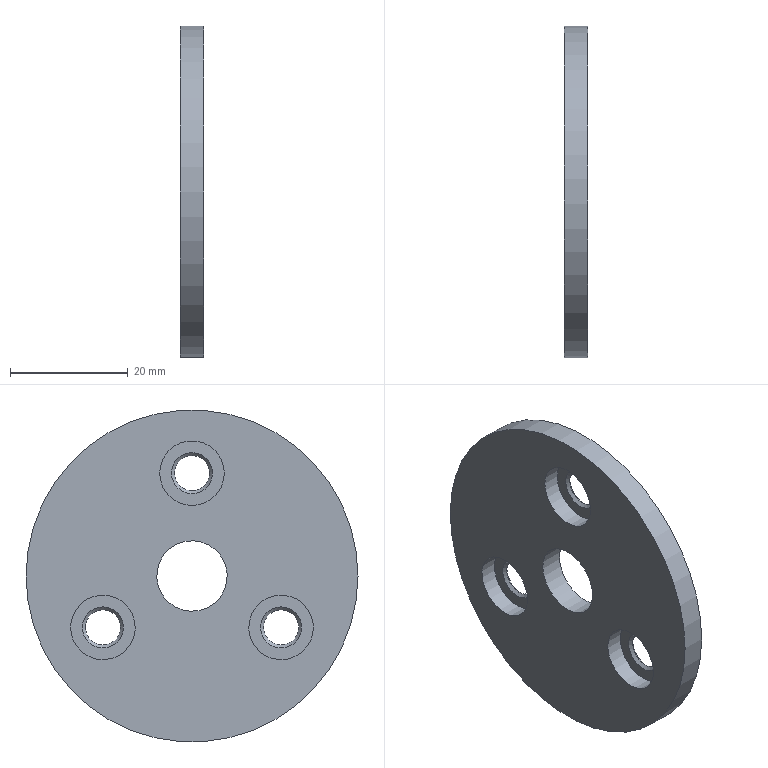Component | NX | FRONT_END_COVER_2 | 1 solid | 16 faces | box 4 x 56.5 x 56.5 mm | volume 8621 mm3 | cone 6 | plane 5 | cylinder 5 | commonest cylinder face diameters 11 x3 56.5 x1 12 x1
STEP:
#1=CARTESIAN_POINT('',(0.,0.,0.));
#2=DIRECTION('',(0.,0.,1.));
#3=DIRECTION('',(1.,0.,0.));
#4=AXIS2_PLACEMENT_3D('',#1,#2,#3);
#5=CARTESIAN_POINT('',(4.,-66.905,79.013));
#6=VERTEX_POINT('',#5);
#7=CARTESIAN_POINT('',(4.,-64.155,74.25));
#8=DIRECTION('',(1.,0.,0.));
#9=DIRECTION('',(0.,-0.5,0.866));
#10=AXIS2_PLACEMENT_3D('',#7,#8,#9);
#11=CIRCLE('',#10,5.5);
#12=CARTESIAN_POINT('',(4.,-49.,83.));
#13=DIRECTION('',(-1.,0.,0.));
#14=DIRECTION('',(0.,-0.5,0.866));
#15=AXIS2_PLACEMENT_3D('',#12,#13,#14);
#16=PLANE('',#15);
#17=CARTESIAN_POINT('',(5.5,-17.5));
#18=CARTESIAN_POINT('',(5.5,-27.026));
#19=CARTESIAN_POINT('',(-2.75,-22.263));
#20=CARTESIAN_POINT('',(-11.,-17.5));
#21=CARTESIAN_POINT('',(-2.75,-12.737));
#22=CARTESIAN_POINT('',(5.5,-7.974));
#23=CARTESIAN_POINT('',(5.5,-17.5));
#24=(BOUNDED_CURVE()B_SPLINE_CURVE(2,(#17,#18,#19,#20,#21,#22,#23),.UNSPECIFIED.,.T.,.F.)B_SPLINE_CURVE_WITH_KNOTS((1,2,2,2,2,1),(-2.094,0.,2.094,4.189,6.283,8.378),.UNSPECIFIED.)CURVE()GEOMETRIC_REPRESENTATION_ITEM()RATIONAL_B_SPLINE_CURVE((1.,0.5,1.,0.5,1.,0.5,1.))REPRESENTATION_ITEM(''));
#25=(GEOMETRIC_REPRESENTATION_CONTEXT(2)PARAMETRIC_REPRESENTATION_CONTEXT()REPRESENTATION_CONTEXT('',''));
#26=DEFINITIONAL_REPRESENTATION('',(#24),#25);
#27=PCURVE('',#16,#26);
#28=CARTESIAN_POINT('',(7.,-64.155,74.25));
#29=DIRECTION('',(-1.,0.,0.));
#30=DIRECTION('',(0.,-0.5,0.866));
#31=AXIS2_PLACEMENT_3D('',#28,#29,#30);
#32=CYLINDRICAL_SURFACE('',#31,5.5);
#33=CARTESIAN_POINT('',(6.283,3.));
#34=DIRECTION('',(-1.,0.));
#35=VECTOR('',#34,1.);
#36=LINE('',#33,#35);
#37=(GEOMETRIC_REPRESENTATION_CONTEXT(2)PARAMETRIC_REPRESENTATION_CONTEXT()REPRESENTATION_CONTEXT('',''));
#38=DEFINITIONAL_REPRESENTATION('',(#36),#37);
#39=PCURVE('',#32,#38);
#40=SURFACE_CURVE('',#11,(#27,#39),.PCURVE_S1.);
#41=EDGE_CURVE('',#6,#6,#40,.T.);
#42=ORIENTED_EDGE('',*,*,#41,.T.);
#43=EDGE_LOOP('',(#42));
#44=FACE_BOUND('',#43,.T.);
#45=CARTESIAN_POINT('',(4.,-36.595,69.487));
#46=VERTEX_POINT('',#45);
#47=CARTESIAN_POINT('',(4.,-33.845,74.25));
#48=DIRECTION('',(1.,0.,0.));
#49=DIRECTION('',(0.,-0.5,-0.866));
#50=AXIS2_PLACEMENT_3D('',#47,#48,#49);
#51=CIRCLE('',#50,5.5);
#52=CARTESIAN_POINT('',(-17.905,3.987));
#53=CARTESIAN_POINT('',(-26.155,8.75));
#54=CARTESIAN_POINT('',(-17.905,13.513));
#55=CARTESIAN_POINT('',(-9.655,18.276));
#56=CARTESIAN_POINT('',(-9.655,8.75));
#57=CARTESIAN_POINT('',(-9.655,-0.7763));
#58=CARTESIAN_POINT('',(-17.905,3.987));
#59=(BOUNDED_CURVE()B_SPLINE_CURVE(2,(#52,#53,#54,#55,#56,#57,#58),.UNSPECIFIED.,.T.,.F.)B_SPLINE_CURVE_WITH_KNOTS((1,2,2,2,2,1),(-2.094,0.,2.094,4.189,6.283,8.378),.UNSPECIFIED.)CURVE()GEOMETRIC_REPRESENTATION_ITEM()RATIONAL_B_SPLINE_CURVE((1.,0.5,1.,0.5,1.,0.5,1.))REPRESENTATION_ITEM(''));
#60=(GEOMETRIC_REPRESENTATION_CONTEXT(2)PARAMETRIC_REPRESENTATION_CONTEXT()REPRESENTATION_CONTEXT('',''));
#61=DEFINITIONAL_REPRESENTATION('',(#59),#60);
#62=PCURVE('',#16,#61);
#63=CARTESIAN_POINT('',(7.,-33.845,74.25));
#64=DIRECTION('',(-1.,0.,0.));
#65=DIRECTION('',(0.,-0.5,0.866));
#66=AXIS2_PLACEMENT_3D('',#63,#64,#65);
#67=CYLINDRICAL_SURFACE('',#66,5.5);
#68=CARTESIAN_POINT('',(10.472,3.));
#69=DIRECTION('',(-1.,0.));
#70=VECTOR('',#69,1.);
#71=LINE('',#68,#70);
#72=(GEOMETRIC_REPRESENTATION_CONTEXT(2)PARAMETRIC_REPRESENTATION_CONTEXT()REPRESENTATION_CONTEXT('',''));
#73=DEFINITIONAL_REPRESENTATION('',(#71),#72);
#74=PCURVE('',#67,#73);
#75=SURFACE_CURVE('',#51,(#62,#74),.PCURVE_S1.);
#76=EDGE_CURVE('',#46,#46,#75,.T.);
#77=ORIENTED_EDGE('',*,*,#76,.T.);
#78=EDGE_LOOP('',(#77));
#79=FACE_BOUND('',#78,.T.);
#80=CARTESIAN_POINT('',(4.,-43.5,100.5));
#81=VERTEX_POINT('',#80);
#82=CARTESIAN_POINT('',(4.,-49.,100.5));
#83=DIRECTION('',(1.,0.,0.));
#84=DIRECTION('',(0.,1.,0.));
#85=AXIS2_PLACEMENT_3D('',#82,#83,#84);
#86=CIRCLE('',#85,5.5);
#87=CARTESIAN_POINT('',(12.405,13.513));
#88=CARTESIAN_POINT('',(20.655,18.276));
#89=CARTESIAN_POINT('',(20.655,8.75));
#90=CARTESIAN_POINT('',(20.655,-0.7763));
#91=CARTESIAN_POINT('',(12.405,3.987));
#92=CARTESIAN_POINT('',(4.155,8.75));
#93=CARTESIAN_POINT('',(12.405,13.513));
#94=(BOUNDED_CURVE()B_SPLINE_CURVE(2,(#87,#88,#89,#90,#91,#92,#93),.UNSPECIFIED.,.T.,.F.)B_SPLINE_CURVE_WITH_KNOTS((1,2,2,2,2,1),(-2.094,0.,2.094,4.189,6.283,8.378),.UNSPECIFIED.)CURVE()GEOMETRIC_REPRESENTATION_ITEM()RATIONAL_B_SPLINE_CURVE((1.,0.5,1.,0.5,1.,0.5,1.))REPRESENTATION_ITEM(''));
#95=(GEOMETRIC_REPRESENTATION_CONTEXT(2)PARAMETRIC_REPRESENTATION_CONTEXT()REPRESENTATION_CONTEXT('',''));
#96=DEFINITIONAL_REPRESENTATION('',(#94),#95);
#97=PCURVE('',#16,#96);
#98=CARTESIAN_POINT('',(7.,-49.,100.5));
#99=DIRECTION('',(-1.,0.,0.));
#100=DIRECTION('',(0.,-0.5,0.866));
#101=AXIS2_PLACEMENT_3D('',#98,#99,#100);
#102=CYLINDRICAL_SURFACE('',#101,5.5);
#103=CARTESIAN_POINT('',(8.378,3.));
#104=DIRECTION('',(-1.,0.));
#105=VECTOR('',#104,1.);
#106=LINE('',#103,#105);
#107=(GEOMETRIC_REPRESENTATION_CONTEXT(2)PARAMETRIC_REPRESENTATION_CONTEXT()REPRESENTATION_CONTEXT('',''));
#108=DEFINITIONAL_REPRESENTATION('',(#106),#107);
#109=PCURVE('',#102,#108);
#110=SURFACE_CURVE('',#86,(#97,#109),.PCURVE_S1.);
#111=EDGE_CURVE('',#81,#81,#110,.T.);
#112=ORIENTED_EDGE('',*,*,#111,.T.);
#113=EDGE_LOOP('',(#112));
#114=FACE_BOUND('',#113,.T.);
#115=CARTESIAN_POINT('',(4.,-52.,88.196));
#116=VERTEX_POINT('',#115);
#117=CARTESIAN_POINT('',(4.,-49.,83.));
#118=DIRECTION('',(-1.,0.,0.));
#119=DIRECTION('',(0.,-0.5,0.866));
#120=AXIS2_PLACEMENT_3D('',#117,#118,#119);
#121=CIRCLE('',#120,6.);
#122=CARTESIAN_POINT('',(0.,0.));
#123=DIRECTION('',(1.,-0.));
#124=AXIS2_PLACEMENT_2D('',#122,#123);
#125=CIRCLE('',#124,6.);
#126=(GEOMETRIC_REPRESENTATION_CONTEXT(2)PARAMETRIC_REPRESENTATION_CONTEXT()REPRESENTATION_CONTEXT('',''));
#127=DEFINITIONAL_REPRESENTATION('',(#125),#126);
#128=PCURVE('',#16,#127);
#129=CARTESIAN_POINT('',(48.,-49.,83.));
#130=DIRECTION('',(-1.,0.,0.));
#131=DIRECTION('',(0.,-0.5,0.866));
#132=AXIS2_PLACEMENT_3D('',#129,#130,#131);
#133=CYLINDRICAL_SURFACE('',#132,6.);
#134=CARTESIAN_POINT('',(0.,44.));
#135=DIRECTION('',(1.,0.));
#136=VECTOR('',#135,1.);
#137=LINE('',#134,#136);
#138=(GEOMETRIC_REPRESENTATION_CONTEXT(2)PARAMETRIC_REPRESENTATION_CONTEXT()REPRESENTATION_CONTEXT('',''));
#139=DEFINITIONAL_REPRESENTATION('',(#137),#138);
#140=PCURVE('',#133,#139);
#141=SURFACE_CURVE('',#121,(#128,#140),.PCURVE_S1.);
#142=EDGE_CURVE('',#116,#116,#141,.T.);
#143=ORIENTED_EDGE('',*,*,#142,.F.);
#144=EDGE_LOOP('',(#143));
#145=FACE_BOUND('',#144,.T.);
#146=CARTESIAN_POINT('',(4.,-63.125,107.465));
#147=VERTEX_POINT('',#146);
#148=CARTESIAN_POINT('',(4.,-49.,83.));
#149=DIRECTION('',(1.,0.,0.));
#150=DIRECTION('',(0.,-0.5,0.866));
#151=AXIS2_PLACEMENT_3D('',#148,#149,#150);
#152=CIRCLE('',#151,28.25);
#153=CARTESIAN_POINT('',(28.25,0.));
#154=CARTESIAN_POINT('',(28.25,-48.93));
#155=CARTESIAN_POINT('',(-14.125,-24.465));
#156=CARTESIAN_POINT('',(-56.5,-0.));
#157=CARTESIAN_POINT('',(-14.125,24.465));
#158=CARTESIAN_POINT('',(28.25,48.93));
#159=CARTESIAN_POINT('',(28.25,0.));
#160=(BOUNDED_CURVE()B_SPLINE_CURVE(2,(#153,#154,#155,#156,#157,#158,#159),.UNSPECIFIED.,.T.,.F.)B_SPLINE_CURVE_WITH_KNOTS((1,2,2,2,2,1),(-2.094,0.,2.094,4.189,6.283,8.378),.UNSPECIFIED.)CURVE()GEOMETRIC_REPRESENTATION_ITEM()RATIONAL_B_SPLINE_CURVE((1.,0.5,1.,0.5,1.,0.5,1.))REPRESENTATION_ITEM(''));
#161=(GEOMETRIC_REPRESENTATION_CONTEXT(2)PARAMETRIC_REPRESENTATION_CONTEXT()REPRESENTATION_CONTEXT('',''));
#162=DEFINITIONAL_REPRESENTATION('',(#160),#161);
#163=PCURVE('',#16,#162);
#164=CARTESIAN_POINT('',(8.,-49.,83.));
#165=DIRECTION('',(-1.,0.,0.));
#166=DIRECTION('',(0.,-0.5,0.866));
#167=AXIS2_PLACEMENT_3D('',#164,#165,#166);
#168=CYLINDRICAL_SURFACE('',#167,28.25);
#169=CARTESIAN_POINT('',(6.283,4.));
#170=DIRECTION('',(-1.,0.));
#171=VECTOR('',#170,1.);
#172=LINE('',#169,#171);
#173=(GEOMETRIC_REPRESENTATION_CONTEXT(2)PARAMETRIC_REPRESENTATION_CONTEXT()REPRESENTATION_CONTEXT('',''));
#174=DEFINITIONAL_REPRESENTATION('',(#172),#173);
#175=PCURVE('',#168,#174);
#176=SURFACE_CURVE('',#152,(#163,#175),.PCURVE_S1.);
#177=EDGE_CURVE('',#147,#147,#176,.T.);
#178=ORIENTED_EDGE('',*,*,#177,.F.);
#179=EDGE_LOOP('',(#178));
#180=FACE_BOUND('',#179,.T.);
#181=ADVANCED_FACE('',(#44,#79,#114,#145,#180),#16,.T.);
#182=CARTESIAN_POINT('',(8.,-47.25,97.469));
#183=VERTEX_POINT('',#182);
#184=CARTESIAN_POINT('',(8.,-49.,100.5));
#185=DIRECTION('',(-1.,0.,0.));
#186=DIRECTION('',(0.,0.5,-0.866));
#187=AXIS2_PLACEMENT_3D('',#184,#185,#186);
#188=CIRCLE('',#187,3.5);
#189=CARTESIAN_POINT('',(8.,-49.,83.));
#190=DIRECTION('',(1.,0.,0.));
#191=DIRECTION('',(0.,0.5,-0.866));
#192=AXIS2_PLACEMENT_3D('',#189,#190,#191);
#193=PLANE('',#192);
#194=CARTESIAN_POINT('',(-11.655,8.75));
#195=CARTESIAN_POINT('',(-11.655,2.688));
#196=CARTESIAN_POINT('',(-16.905,5.719));
#197=CARTESIAN_POINT('',(-22.155,8.75));
#198=CARTESIAN_POINT('',(-16.905,11.781));
#199=CARTESIAN_POINT('',(-11.655,14.812));
#200=CARTESIAN_POINT('',(-11.655,8.75));
#201=(BOUNDED_CURVE()B_SPLINE_CURVE(2,(#194,#195,#196,#197,#198,#199,#200),.UNSPECIFIED.,.T.,.F.)B_SPLINE_CURVE_WITH_KNOTS((1,2,2,2,2,1),(-2.094,0.,2.094,4.189,6.283,8.378),.UNSPECIFIED.)CURVE()GEOMETRIC_REPRESENTATION_ITEM()RATIONAL_B_SPLINE_CURVE((1.,0.5,1.,0.5,1.,0.5,1.))REPRESENTATION_ITEM(''));
#202=(GEOMETRIC_REPRESENTATION_CONTEXT(2)PARAMETRIC_REPRESENTATION_CONTEXT()REPRESENTATION_CONTEXT('',''));
#203=DEFINITIONAL_REPRESENTATION('',(#201),#202);
#204=PCURVE('',#193,#203);
#205=CARTESIAN_POINT('',(7.5,-49.,100.5));
#206=DIRECTION('',(1.,0.,0.));
#207=DIRECTION('',(0.,0.5,-0.866));
#208=AXIS2_PLACEMENT_3D('',#205,#206,#207);
#209=CONICAL_SURFACE('',#208,3.,0.7854);
#210=CARTESIAN_POINT('',(6.283,0.5));
#211=DIRECTION('',(-1.,0.));
#212=VECTOR('',#211,1.);
#213=LINE('',#210,#212);
#214=(GEOMETRIC_REPRESENTATION_CONTEXT(2)PARAMETRIC_REPRESENTATION_CONTEXT()REPRESENTATION_CONTEXT('',''));
#215=DEFINITIONAL_REPRESENTATION('',(#213),#214);
#216=PCURVE('',#209,#215);
#217=SURFACE_CURVE('',#188,(#204,#216),.PCURVE_S1.);
#218=EDGE_CURVE('',#183,#183,#217,.T.);
#219=ORIENTED_EDGE('',*,*,#218,.T.);
#220=EDGE_LOOP('',(#219));
#221=FACE_BOUND('',#220,.T.);
#222=CARTESIAN_POINT('',(8.,-62.405,71.219));
#223=VERTEX_POINT('',#222);
#224=CARTESIAN_POINT('',(8.,-64.155,74.25));
#225=DIRECTION('',(-1.,0.,0.));
#226=DIRECTION('',(0.,0.5,-0.866));
#227=AXIS2_PLACEMENT_3D('',#224,#225,#226);
#228=CIRCLE('',#227,3.5);
#229=CARTESIAN_POINT('',(3.5,-17.5));
#230=CARTESIAN_POINT('',(3.5,-23.562));
#231=CARTESIAN_POINT('',(-1.75,-20.531));
#232=CARTESIAN_POINT('',(-7.,-17.5));
#233=CARTESIAN_POINT('',(-1.75,-14.469));
#234=CARTESIAN_POINT('',(3.5,-11.438));
#235=CARTESIAN_POINT('',(3.5,-17.5));
#236=(BOUNDED_CURVE()B_SPLINE_CURVE(2,(#229,#230,#231,#232,#233,#234,#235),.UNSPECIFIED.,.T.,.F.)B_SPLINE_CURVE_WITH_KNOTS((1,2,2,2,2,1),(-2.094,0.,2.094,4.189,6.283,8.378),.UNSPECIFIED.)CURVE()GEOMETRIC_REPRESENTATION_ITEM()RATIONAL_B_SPLINE_CURVE((1.,0.5,1.,0.5,1.,0.5,1.))REPRESENTATION_ITEM(''));
#237=(GEOMETRIC_REPRESENTATION_CONTEXT(2)PARAMETRIC_REPRESENTATION_CONTEXT()REPRESENTATION_CONTEXT('',''));
#238=DEFINITIONAL_REPRESENTATION('',(#236),#237);
#239=PCURVE('',#193,#238);
#240=CARTESIAN_POINT('',(7.5,-64.155,74.25));
#241=DIRECTION('',(1.,0.,0.));
#242=DIRECTION('',(0.,0.5,-0.866));
#243=AXIS2_PLACEMENT_3D('',#240,#241,#242);
#244=CONICAL_SURFACE('',#243,3.,0.7854);
#245=CARTESIAN_POINT('',(6.283,0.5));
#246=DIRECTION('',(-1.,0.));
#247=VECTOR('',#246,1.);
#248=LINE('',#245,#247);
#249=(GEOMETRIC_REPRESENTATION_CONTEXT(2)PARAMETRIC_REPRESENTATION_CONTEXT()REPRESENTATION_CONTEXT('',''));
#250=DEFINITIONAL_REPRESENTATION('',(#248),#249);
#251=PCURVE('',#244,#250);
#252=SURFACE_CURVE('',#228,(#239,#251),.PCURVE_S1.);
#253=EDGE_CURVE('',#223,#223,#252,.T.);
#254=ORIENTED_EDGE('',*,*,#253,.T.);
#255=EDGE_LOOP('',(#254));
#256=FACE_BOUND('',#255,.T.);
#257=CARTESIAN_POINT('',(8.,-32.095,71.219));
#258=VERTEX_POINT('',#257);
#259=CARTESIAN_POINT('',(8.,-33.845,74.25));
#260=DIRECTION('',(-1.,0.,0.));
#261=DIRECTION('',(0.,0.5,-0.866));
#262=AXIS2_PLACEMENT_3D('',#259,#260,#261);
#263=CIRCLE('',#262,3.5);
#264=CARTESIAN_POINT('',(18.655,8.75));
#265=CARTESIAN_POINT('',(18.655,2.688));
#266=CARTESIAN_POINT('',(13.405,5.719));
#267=CARTESIAN_POINT('',(8.155,8.75));
#268=CARTESIAN_POINT('',(13.405,11.781));
#269=CARTESIAN_POINT('',(18.655,14.812));
#270=CARTESIAN_POINT('',(18.655,8.75));
#271=(BOUNDED_CURVE()B_SPLINE_CURVE(2,(#264,#265,#266,#267,#268,#269,#270),.UNSPECIFIED.,.T.,.F.)B_SPLINE_CURVE_WITH_KNOTS((1,2,2,2,2,1),(-2.094,0.,2.094,4.189,6.283,8.378),.UNSPECIFIED.)CURVE()GEOMETRIC_REPRESENTATION_ITEM()RATIONAL_B_SPLINE_CURVE((1.,0.5,1.,0.5,1.,0.5,1.))REPRESENTATION_ITEM(''));
#272=(GEOMETRIC_REPRESENTATION_CONTEXT(2)PARAMETRIC_REPRESENTATION_CONTEXT()REPRESENTATION_CONTEXT('',''));
#273=DEFINITIONAL_REPRESENTATION('',(#271),#272);
#274=PCURVE('',#193,#273);
#275=CARTESIAN_POINT('',(7.5,-33.845,74.25));
#276=DIRECTION('',(1.,0.,0.));
#277=DIRECTION('',(0.,0.5,-0.866));
#278=AXIS2_PLACEMENT_3D('',#275,#276,#277);
#279=CONICAL_SURFACE('',#278,3.,0.7854);
#280=CARTESIAN_POINT('',(6.283,0.5));
#281=DIRECTION('',(-1.,-0.));
#282=VECTOR('',#281,1.);
#283=LINE('',#280,#282);
#284=(GEOMETRIC_REPRESENTATION_CONTEXT(2)PARAMETRIC_REPRESENTATION_CONTEXT()REPRESENTATION_CONTEXT('',''));
#285=DEFINITIONAL_REPRESENTATION('',(#283),#284);
#286=PCURVE('',#279,#285);
#287=SURFACE_CURVE('',#263,(#274,#286),.PCURVE_S1.);
#288=EDGE_CURVE('',#258,#258,#287,.T.);
#289=ORIENTED_EDGE('',*,*,#288,.T.);
#290=EDGE_LOOP('',(#289));
#291=FACE_BOUND('',#290,.T.);
#292=CARTESIAN_POINT('',(8.,-46.,77.804));
#293=VERTEX_POINT('',#292);
#294=CARTESIAN_POINT('',(8.,-52.,88.196));
#295=VERTEX_POINT('',#294);
#296=CARTESIAN_POINT('',(8.,-49.,83.));
#297=DIRECTION('',(1.,0.,0.));
#298=DIRECTION('',(0.,0.5,-0.866));
#299=AXIS2_PLACEMENT_3D('',#296,#297,#298);
#300=CIRCLE('',#299,6.);
#301=CARTESIAN_POINT('',(0.,0.));
#302=DIRECTION('',(1.,0.));
#303=AXIS2_PLACEMENT_2D('',#301,#302);
#304=CIRCLE('',#303,6.);
#305=(GEOMETRIC_REPRESENTATION_CONTEXT(2)PARAMETRIC_REPRESENTATION_CONTEXT()REPRESENTATION_CONTEXT('',''));
#306=DEFINITIONAL_REPRESENTATION('',(#304),#305);
#307=PCURVE('',#193,#306);
#308=CARTESIAN_POINT('',(3.142,40.));
#309=DIRECTION('',(-1.,0.));
#310=VECTOR('',#309,1.);
#311=LINE('',#308,#310);
#312=(GEOMETRIC_REPRESENTATION_CONTEXT(2)PARAMETRIC_REPRESENTATION_CONTEXT()REPRESENTATION_CONTEXT('',''));
#313=DEFINITIONAL_REPRESENTATION('',(#311),#312);
#314=PCURVE('',#133,#313);
#315=SURFACE_CURVE('',#300,(#307,#314),.PCURVE_S1.);
#316=EDGE_CURVE('',#293,#295,#315,.T.);
#317=ORIENTED_EDGE('',*,*,#316,.F.);
#318=CARTESIAN_POINT('',(8.,-49.,83.));
#319=DIRECTION('',(1.,0.,0.));
#320=DIRECTION('',(0.,0.5,-0.866));
#321=AXIS2_PLACEMENT_3D('',#318,#319,#320);
#322=CIRCLE('',#321,6.);
#323=CARTESIAN_POINT('',(0.,0.));
#324=DIRECTION('',(1.,0.));
#325=AXIS2_PLACEMENT_2D('',#323,#324);
#326=CIRCLE('',#325,6.);
#327=(GEOMETRIC_REPRESENTATION_CONTEXT(2)PARAMETRIC_REPRESENTATION_CONTEXT()REPRESENTATION_CONTEXT('',''));
#328=DEFINITIONAL_REPRESENTATION('',(#326),#327);
#329=PCURVE('',#193,#328);
#330=CARTESIAN_POINT('',(9.425,40.));
#331=DIRECTION('',(-1.,0.));
#332=VECTOR('',#331,1.);
#333=LINE('',#330,#332);
#334=(GEOMETRIC_REPRESENTATION_CONTEXT(2)PARAMETRIC_REPRESENTATION_CONTEXT()REPRESENTATION_CONTEXT('',''));
#335=DEFINITIONAL_REPRESENTATION('',(#333),#334);
#336=PCURVE('',#133,#335);
#337=SURFACE_CURVE('',#322,(#329,#336),.PCURVE_S1.);
#338=EDGE_CURVE('',#295,#293,#337,.T.);
#339=ORIENTED_EDGE('',*,*,#338,.F.);
#340=EDGE_LOOP('',(#317,#339));
#341=FACE_BOUND('',#340,.T.);
#342=CARTESIAN_POINT('',(8.,-63.125,107.465));
#343=VERTEX_POINT('',#342);
#344=CARTESIAN_POINT('',(8.,-49.,83.));
#345=DIRECTION('',(-1.,0.,0.));
#346=DIRECTION('',(0.,-0.5,0.866));
#347=AXIS2_PLACEMENT_3D('',#344,#345,#346);
#348=CIRCLE('',#347,28.25);
#349=CARTESIAN_POINT('',(-28.25,0.));
#350=CARTESIAN_POINT('',(-28.25,48.93));
#351=CARTESIAN_POINT('',(14.125,24.465));
#352=CARTESIAN_POINT('',(56.5,0.));
#353=CARTESIAN_POINT('',(14.125,-24.465));
#354=CARTESIAN_POINT('',(-28.25,-48.93));
#355=CARTESIAN_POINT('',(-28.25,0.));
#356=(BOUNDED_CURVE()B_SPLINE_CURVE(2,(#349,#350,#351,#352,#353,#354,#355),.UNSPECIFIED.,.T.,.F.)B_SPLINE_CURVE_WITH_KNOTS((1,2,2,2,2,1),(-2.094,0.,2.094,4.189,6.283,8.378),.UNSPECIFIED.)CURVE()GEOMETRIC_REPRESENTATION_ITEM()RATIONAL_B_SPLINE_CURVE((1.,0.5,1.,0.5,1.,0.5,1.))REPRESENTATION_ITEM(''));
#357=(GEOMETRIC_REPRESENTATION_CONTEXT(2)PARAMETRIC_REPRESENTATION_CONTEXT()REPRESENTATION_CONTEXT('',''));
#358=DEFINITIONAL_REPRESENTATION('',(#356),#357);
#359=PCURVE('',#193,#358);
#360=CARTESIAN_POINT('',(0.,0.));
#361=DIRECTION('',(1.,0.));
#362=VECTOR('',#361,1.);
#363=LINE('',#360,#362);
#364=(GEOMETRIC_REPRESENTATION_CONTEXT(2)PARAMETRIC_REPRESENTATION_CONTEXT()REPRESENTATION_CONTEXT('',''));
#365=DEFINITIONAL_REPRESENTATION('',(#363),#364);
#366=PCURVE('',#168,#365);
#367=SURFACE_CURVE('',#348,(#359,#366),.PCURVE_S1.);
#368=EDGE_CURVE('',#343,#343,#367,.T.);
#369=ORIENTED_EDGE('',*,*,#368,.F.);
#370=EDGE_LOOP('',(#369));
#371=FACE_BOUND('',#370,.T.);
#372=ADVANCED_FACE('',(#221,#256,#291,#341,#371),#193,.T.);
#373=ORIENTED_EDGE('',*,*,#177,.T.);
#374=CARTESIAN_POINT('',(8.,-63.125,107.465));
#375=CARTESIAN_POINT('',(4.,-63.125,107.465));
#376=B_SPLINE_CURVE_WITH_KNOTS('',1,(#374,#375),.UNSPECIFIED.,.F.,.F.,(2,2),(0.,4.),.PIECEWISE_BEZIER_KNOTS.);
#377=CARTESIAN_POINT('',(0.,0.));
#378=DIRECTION('',(0.,1.));
#379=VECTOR('',#378,1.);
#380=LINE('',#377,#379);
#381=(GEOMETRIC_REPRESENTATION_CONTEXT(2)PARAMETRIC_REPRESENTATION_CONTEXT()REPRESENTATION_CONTEXT('',''));
#382=DEFINITIONAL_REPRESENTATION('',(#380),#381);
#383=PCURVE('',#168,#382);
#384=CARTESIAN_POINT('',(6.283,0.));
#385=DIRECTION('',(0.,1.));
#386=VECTOR('',#385,1.);
#387=LINE('',#384,#386);
#388=(GEOMETRIC_REPRESENTATION_CONTEXT(2)PARAMETRIC_REPRESENTATION_CONTEXT()REPRESENTATION_CONTEXT('',''));
#389=DEFINITIONAL_REPRESENTATION('',(#387),#388);
#390=PCURVE('',#168,#389);
#391=SEAM_CURVE('',#376,(#383,#390),.PCURVE_S1.);
#392=EDGE_CURVE('',#343,#147,#391,.T.);
#393=ORIENTED_EDGE('',*,*,#392,.F.);
#394=ORIENTED_EDGE('',*,*,#368,.T.);
#395=ORIENTED_EDGE('',*,*,#392,.T.);
#396=EDGE_LOOP('',(#373,#393,#394,#395));
#397=FACE_BOUND('',#396,.T.);
#398=ADVANCED_FACE('',(#397),#168,.T.);
#399=ORIENTED_EDGE('',*,*,#338,.F.);
#400=CARTESIAN_POINT('',(8.,-52.,88.196));
#401=CARTESIAN_POINT('',(4.,-52.,88.196));
#402=B_SPLINE_CURVE_WITH_KNOTS('',1,(#400,#401),.UNSPECIFIED.,.F.,.F.,(2,2),(40.,44.),.PIECEWISE_BEZIER_KNOTS.);
#403=CARTESIAN_POINT('',(6.283,0.));
#404=DIRECTION('',(0.,1.));
#405=VECTOR('',#404,1.);
#406=LINE('',#403,#405);
#407=(GEOMETRIC_REPRESENTATION_CONTEXT(2)PARAMETRIC_REPRESENTATION_CONTEXT()REPRESENTATION_CONTEXT('',''));
#408=DEFINITIONAL_REPRESENTATION('',(#406),#407);
#409=PCURVE('',#133,#408);
#410=CARTESIAN_POINT('',(0.,0.));
#411=DIRECTION('',(0.,1.));
#412=VECTOR('',#411,1.);
#413=LINE('',#410,#412);
#414=(GEOMETRIC_REPRESENTATION_CONTEXT(2)PARAMETRIC_REPRESENTATION_CONTEXT()REPRESENTATION_CONTEXT('',''));
#415=DEFINITIONAL_REPRESENTATION('',(#413),#414);
#416=PCURVE('',#133,#415);
#417=SEAM_CURVE('',#402,(#409,#416),.PCURVE_S1.);
#418=EDGE_CURVE('',#295,#116,#417,.T.);
#419=ORIENTED_EDGE('',*,*,#418,.T.);
#420=ORIENTED_EDGE('',*,*,#142,.F.);
#421=ORIENTED_EDGE('',*,*,#418,.F.);
#422=ORIENTED_EDGE('',*,*,#316,.F.);
#423=EDGE_LOOP('',(#399,#419,#420,#421,#422));
#424=FACE_BOUND('',#423,.F.);
#425=ADVANCED_FACE('',(#424),#133,.F.);
#426=CARTESIAN_POINT('',(7.,-43.5,100.5));
#427=VERTEX_POINT('',#426);
#428=CARTESIAN_POINT('',(7.,-49.,100.5));
#429=DIRECTION('',(-1.,0.,0.));
#430=DIRECTION('',(0.,1.,0.));
#431=AXIS2_PLACEMENT_3D('',#428,#429,#430);
#432=CIRCLE('',#431,5.5);
#433=CARTESIAN_POINT('',(2.094,0.));
#434=DIRECTION('',(1.,0.));
#435=VECTOR('',#434,1.);
#436=LINE('',#433,#435);
#437=(GEOMETRIC_REPRESENTATION_CONTEXT(2)PARAMETRIC_REPRESENTATION_CONTEXT()REPRESENTATION_CONTEXT('',''));
#438=DEFINITIONAL_REPRESENTATION('',(#436),#437);
#439=PCURVE('',#102,#438);
#440=CARTESIAN_POINT('',(7.,-49.,100.5));
#441=DIRECTION('',(1.,0.,0.));
#442=DIRECTION('',(0.,0.5,-0.866));
#443=AXIS2_PLACEMENT_3D('',#440,#441,#442);
#444=PLANE('',#443);
#445=CARTESIAN_POINT('',(2.75,4.763));
#446=CARTESIAN_POINT('',(11.,0.));
#447=CARTESIAN_POINT('',(2.75,-4.763));
#448=CARTESIAN_POINT('',(-5.5,-9.526));
#449=CARTESIAN_POINT('',(-5.5,-0.));
#450=CARTESIAN_POINT('',(-5.5,9.526));
#451=CARTESIAN_POINT('',(2.75,4.763));
#452=(BOUNDED_CURVE()B_SPLINE_CURVE(2,(#445,#446,#447,#448,#449,#450,#451),.UNSPECIFIED.,.T.,.F.)B_SPLINE_CURVE_WITH_KNOTS((1,2,2,2,2,1),(-2.094,0.,2.094,4.189,6.283,8.378),.UNSPECIFIED.)CURVE()GEOMETRIC_REPRESENTATION_ITEM()RATIONAL_B_SPLINE_CURVE((1.,0.5,1.,0.5,1.,0.5,1.))REPRESENTATION_ITEM(''));
#453=(GEOMETRIC_REPRESENTATION_CONTEXT(2)PARAMETRIC_REPRESENTATION_CONTEXT()REPRESENTATION_CONTEXT('',''));
#454=DEFINITIONAL_REPRESENTATION('',(#452),#453);
#455=PCURVE('',#444,#454);
#456=SURFACE_CURVE('',#432,(#439,#455),.PCURVE_S1.);
#457=EDGE_CURVE('',#427,#427,#456,.T.);
#458=ORIENTED_EDGE('',*,*,#457,.T.);
#459=CARTESIAN_POINT('',(7.,-43.5,100.5));
#460=CARTESIAN_POINT('',(4.,-43.5,100.5));
#461=B_SPLINE_CURVE_WITH_KNOTS('',1,(#459,#460),.UNSPECIFIED.,.F.,.F.,(2,2),(0.,3.),.PIECEWISE_BEZIER_KNOTS.);
#462=CARTESIAN_POINT('',(8.378,0.));
#463=DIRECTION('',(0.,1.));
#464=VECTOR('',#463,1.);
#465=LINE('',#462,#464);
#466=(GEOMETRIC_REPRESENTATION_CONTEXT(2)PARAMETRIC_REPRESENTATION_CONTEXT()REPRESENTATION_CONTEXT('',''));
#467=DEFINITIONAL_REPRESENTATION('',(#465),#466);
#468=PCURVE('',#102,#467);
#469=CARTESIAN_POINT('',(2.094,0.));
#470=DIRECTION('',(0.,1.));
#471=VECTOR('',#470,1.);
#472=LINE('',#469,#471);
#473=(GEOMETRIC_REPRESENTATION_CONTEXT(2)PARAMETRIC_REPRESENTATION_CONTEXT()REPRESENTATION_CONTEXT('',''));
#474=DEFINITIONAL_REPRESENTATION('',(#472),#473);
#475=PCURVE('',#102,#474);
#476=SEAM_CURVE('',#461,(#468,#475),.PCURVE_S1.);
#477=EDGE_CURVE('',#427,#81,#476,.T.);
#478=ORIENTED_EDGE('',*,*,#477,.T.);
#479=ORIENTED_EDGE('',*,*,#111,.T.);
#480=ORIENTED_EDGE('',*,*,#477,.F.);
#481=EDGE_LOOP('',(#458,#478,#479,#480));
#482=FACE_BOUND('',#481,.F.);
#483=ADVANCED_FACE('',(#482),#102,.F.);
#484=CARTESIAN_POINT('',(7.,-47.25,97.469));
#485=VERTEX_POINT('',#484);
#486=CARTESIAN_POINT('',(7.,-49.,100.5));
#487=DIRECTION('',(1.,0.,0.));
#488=DIRECTION('',(0.,0.5,-0.866));
#489=AXIS2_PLACEMENT_3D('',#486,#487,#488);
#490=CIRCLE('',#489,3.5);
#491=CARTESIAN_POINT('',(0.,0.));
#492=DIRECTION('',(1.,-0.));
#493=AXIS2_PLACEMENT_2D('',#491,#492);
#494=CIRCLE('',#493,3.5);
#495=(GEOMETRIC_REPRESENTATION_CONTEXT(2)PARAMETRIC_REPRESENTATION_CONTEXT()REPRESENTATION_CONTEXT('',''));
#496=DEFINITIONAL_REPRESENTATION('',(#494),#495);
#497=PCURVE('',#444,#496);
#498=CARTESIAN_POINT('',(7.,-49.,100.5));
#499=DIRECTION('',(-1.,0.,0.));
#500=DIRECTION('',(0.,-0.5,0.866));
#501=AXIS2_PLACEMENT_3D('',#498,#499,#500);
#502=CONICAL_SURFACE('',#501,3.5,0.7854);
#503=CARTESIAN_POINT('',(9.425,0.));
#504=DIRECTION('',(-1.,0.));
#505=VECTOR('',#504,1.);
#506=LINE('',#503,#505);
#507=(GEOMETRIC_REPRESENTATION_CONTEXT(2)PARAMETRIC_REPRESENTATION_CONTEXT()REPRESENTATION_CONTEXT('',''));
#508=DEFINITIONAL_REPRESENTATION('',(#506),#507);
#509=PCURVE('',#502,#508);
#510=SURFACE_CURVE('',#490,(#497,#509),.PCURVE_S1.);
#511=EDGE_CURVE('',#485,#485,#510,.T.);
#512=ORIENTED_EDGE('',*,*,#511,.T.);
#513=EDGE_LOOP('',(#512));
#514=FACE_BOUND('',#513,.T.);
#515=ORIENTED_EDGE('',*,*,#457,.T.);
#516=EDGE_LOOP('',(#515));
#517=FACE_BOUND('',#516,.T.);
#518=ADVANCED_FACE('',(#514,#517),#444,.F.);
#519=CARTESIAN_POINT('',(7.,-36.595,69.487));
#520=VERTEX_POINT('',#519);
#521=CARTESIAN_POINT('',(7.,-33.845,74.25));
#522=DIRECTION('',(-1.,0.,0.));
#523=DIRECTION('',(0.,-0.5,-0.866));
#524=AXIS2_PLACEMENT_3D('',#521,#522,#523);
#525=CIRCLE('',#524,5.5);
#526=CARTESIAN_POINT('',(4.189,0.));
#527=DIRECTION('',(1.,0.));
#528=VECTOR('',#527,1.);
#529=LINE('',#526,#528);
#530=(GEOMETRIC_REPRESENTATION_CONTEXT(2)PARAMETRIC_REPRESENTATION_CONTEXT()REPRESENTATION_CONTEXT('',''));
#531=DEFINITIONAL_REPRESENTATION('',(#529),#530);
#532=PCURVE('',#67,#531);
#533=CARTESIAN_POINT('',(7.,-33.845,74.25));
#534=DIRECTION('',(1.,0.,0.));
#535=DIRECTION('',(0.,0.5,-0.866));
#536=AXIS2_PLACEMENT_3D('',#533,#534,#535);
#537=PLANE('',#536);
#538=CARTESIAN_POINT('',(2.75,-4.763));
#539=CARTESIAN_POINT('',(-5.5,-9.526));
#540=CARTESIAN_POINT('',(-5.5,-0.));
#541=CARTESIAN_POINT('',(-5.5,9.526));
#542=CARTESIAN_POINT('',(2.75,4.763));
#543=CARTESIAN_POINT('',(11.,0.));
#544=CARTESIAN_POINT('',(2.75,-4.763));
#545=(BOUNDED_CURVE()B_SPLINE_CURVE(2,(#538,#539,#540,#541,#542,#543,#544),.UNSPECIFIED.,.T.,.F.)B_SPLINE_CURVE_WITH_KNOTS((1,2,2,2,2,1),(-2.094,0.,2.094,4.189,6.283,8.378),.UNSPECIFIED.)CURVE()GEOMETRIC_REPRESENTATION_ITEM()RATIONAL_B_SPLINE_CURVE((1.,0.5,1.,0.5,1.,0.5,1.))REPRESENTATION_ITEM(''));
#546=(GEOMETRIC_REPRESENTATION_CONTEXT(2)PARAMETRIC_REPRESENTATION_CONTEXT()REPRESENTATION_CONTEXT('',''));
#547=DEFINITIONAL_REPRESENTATION('',(#545),#546);
#548=PCURVE('',#537,#547);
#549=SURFACE_CURVE('',#525,(#532,#548),.PCURVE_S1.);
#550=EDGE_CURVE('',#520,#520,#549,.T.);
#551=ORIENTED_EDGE('',*,*,#550,.T.);
#552=CARTESIAN_POINT('',(7.,-36.595,69.487));
#553=CARTESIAN_POINT('',(4.,-36.595,69.487));
#554=B_SPLINE_CURVE_WITH_KNOTS('',1,(#552,#553),.UNSPECIFIED.,.F.,.F.,(2,2),(0.,3.),.PIECEWISE_BEZIER_KNOTS.);
#555=CARTESIAN_POINT('',(10.472,0.));
#556=DIRECTION('',(0.,1.));
#557=VECTOR('',#556,1.);
#558=LINE('',#555,#557);
#559=(GEOMETRIC_REPRESENTATION_CONTEXT(2)PARAMETRIC_REPRESENTATION_CONTEXT()REPRESENTATION_CONTEXT('',''));
#560=DEFINITIONAL_REPRESENTATION('',(#558),#559);
#561=PCURVE('',#67,#560);
#562=CARTESIAN_POINT('',(4.189,0.));
#563=DIRECTION('',(0.,1.));
#564=VECTOR('',#563,1.);
#565=LINE('',#562,#564);
#566=(GEOMETRIC_REPRESENTATION_CONTEXT(2)PARAMETRIC_REPRESENTATION_CONTEXT()REPRESENTATION_CONTEXT('',''));
#567=DEFINITIONAL_REPRESENTATION('',(#565),#566);
#568=PCURVE('',#67,#567);
#569=SEAM_CURVE('',#554,(#561,#568),.PCURVE_S1.);
#570=EDGE_CURVE('',#520,#46,#569,.T.);
#571=ORIENTED_EDGE('',*,*,#570,.T.);
#572=ORIENTED_EDGE('',*,*,#76,.T.);
#573=ORIENTED_EDGE('',*,*,#570,.F.);
#574=EDGE_LOOP('',(#551,#571,#572,#573));
#575=FACE_BOUND('',#574,.F.);
#576=ADVANCED_FACE('',(#575),#67,.F.);
#577=CARTESIAN_POINT('',(7.,-32.095,71.219));
#578=VERTEX_POINT('',#577);
#579=CARTESIAN_POINT('',(7.,-33.845,74.25));
#580=DIRECTION('',(1.,0.,0.));
#581=DIRECTION('',(0.,0.5,-0.866));
#582=AXIS2_PLACEMENT_3D('',#579,#580,#581);
#583=CIRCLE('',#582,3.5);
#584=CARTESIAN_POINT('',(0.,0.));
#585=DIRECTION('',(1.,-0.));
#586=AXIS2_PLACEMENT_2D('',#584,#585);
#587=CIRCLE('',#586,3.5);
#588=(GEOMETRIC_REPRESENTATION_CONTEXT(2)PARAMETRIC_REPRESENTATION_CONTEXT()REPRESENTATION_CONTEXT('',''));
#589=DEFINITIONAL_REPRESENTATION('',(#587),#588);
#590=PCURVE('',#537,#589);
#591=CARTESIAN_POINT('',(7.,-33.845,74.25));
#592=DIRECTION('',(-1.,0.,0.));
#593=DIRECTION('',(0.,-0.5,0.866));
#594=AXIS2_PLACEMENT_3D('',#591,#592,#593);
#595=CONICAL_SURFACE('',#594,3.5,0.7854);
#596=CARTESIAN_POINT('',(9.425,0.));
#597=DIRECTION('',(-1.,0.));
#598=VECTOR('',#597,1.);
#599=LINE('',#596,#598);
#600=(GEOMETRIC_REPRESENTATION_CONTEXT(2)PARAMETRIC_REPRESENTATION_CONTEXT()REPRESENTATION_CONTEXT('',''));
#601=DEFINITIONAL_REPRESENTATION('',(#599),#600);
#602=PCURVE('',#595,#601);
#603=SURFACE_CURVE('',#583,(#590,#602),.PCURVE_S1.);
#604=EDGE_CURVE('',#578,#578,#603,.T.);
#605=ORIENTED_EDGE('',*,*,#604,.T.);
#606=EDGE_LOOP('',(#605));
#607=FACE_BOUND('',#606,.T.);
#608=ORIENTED_EDGE('',*,*,#550,.T.);
#609=EDGE_LOOP('',(#608));
#610=FACE_BOUND('',#609,.T.);
#611=ADVANCED_FACE('',(#607,#610),#537,.F.);
#612=CARTESIAN_POINT('',(7.,-66.905,79.013));
#613=VERTEX_POINT('',#612);
#614=CARTESIAN_POINT('',(7.,-64.155,74.25));
#615=DIRECTION('',(-1.,0.,0.));
#616=DIRECTION('',(0.,-0.5,0.866));
#617=AXIS2_PLACEMENT_3D('',#614,#615,#616);
#618=CIRCLE('',#617,5.5);
#619=CARTESIAN_POINT('',(0.,0.));
#620=DIRECTION('',(1.,0.));
#621=VECTOR('',#620,1.);
#622=LINE('',#619,#621);
#623=(GEOMETRIC_REPRESENTATION_CONTEXT(2)PARAMETRIC_REPRESENTATION_CONTEXT()REPRESENTATION_CONTEXT('',''));
#624=DEFINITIONAL_REPRESENTATION('',(#622),#623);
#625=PCURVE('',#32,#624);
#626=CARTESIAN_POINT('',(7.,-64.155,74.25));
#627=DIRECTION('',(1.,0.,0.));
#628=DIRECTION('',(0.,0.5,-0.866));
#629=AXIS2_PLACEMENT_3D('',#626,#627,#628);
#630=PLANE('',#629);
#631=CARTESIAN_POINT('',(-5.5,0.));
#632=CARTESIAN_POINT('',(-5.5,9.526));
#633=CARTESIAN_POINT('',(2.75,4.763));
#634=CARTESIAN_POINT('',(11.,-0.));
#635=CARTESIAN_POINT('',(2.75,-4.763));
#636=CARTESIAN_POINT('',(-5.5,-9.526));
#637=CARTESIAN_POINT('',(-5.5,0.));
#638=(BOUNDED_CURVE()B_SPLINE_CURVE(2,(#631,#632,#633,#634,#635,#636,#637),.UNSPECIFIED.,.T.,.F.)B_SPLINE_CURVE_WITH_KNOTS((1,2,2,2,2,1),(-2.094,0.,2.094,4.189,6.283,8.378),.UNSPECIFIED.)CURVE()GEOMETRIC_REPRESENTATION_ITEM()RATIONAL_B_SPLINE_CURVE((1.,0.5,1.,0.5,1.,0.5,1.))REPRESENTATION_ITEM(''));
#639=(GEOMETRIC_REPRESENTATION_CONTEXT(2)PARAMETRIC_REPRESENTATION_CONTEXT()REPRESENTATION_CONTEXT('',''));
#640=DEFINITIONAL_REPRESENTATION('',(#638),#639);
#641=PCURVE('',#630,#640);
#642=SURFACE_CURVE('',#618,(#625,#641),.PCURVE_S1.);
#643=EDGE_CURVE('',#613,#613,#642,.T.);
#644=ORIENTED_EDGE('',*,*,#643,.T.);
#645=CARTESIAN_POINT('',(7.,-66.905,79.013));
#646=CARTESIAN_POINT('',(4.,-66.905,79.013));
#647=B_SPLINE_CURVE_WITH_KNOTS('',1,(#645,#646),.UNSPECIFIED.,.F.,.F.,(2,2),(0.,3.),.PIECEWISE_BEZIER_KNOTS.);
#648=CARTESIAN_POINT('',(6.283,0.));
#649=DIRECTION('',(0.,1.));
#650=VECTOR('',#649,1.);
#651=LINE('',#648,#650);
#652=(GEOMETRIC_REPRESENTATION_CONTEXT(2)PARAMETRIC_REPRESENTATION_CONTEXT()REPRESENTATION_CONTEXT('',''));
#653=DEFINITIONAL_REPRESENTATION('',(#651),#652);
#654=PCURVE('',#32,#653);
#655=CARTESIAN_POINT('',(0.,0.));
#656=DIRECTION('',(0.,1.));
#657=VECTOR('',#656,1.);
#658=LINE('',#655,#657);
#659=(GEOMETRIC_REPRESENTATION_CONTEXT(2)PARAMETRIC_REPRESENTATION_CONTEXT()REPRESENTATION_CONTEXT('',''));
#660=DEFINITIONAL_REPRESENTATION('',(#658),#659);
#661=PCURVE('',#32,#660);
#662=SEAM_CURVE('',#647,(#654,#661),.PCURVE_S1.);
#663=EDGE_CURVE('',#613,#6,#662,.T.);
#664=ORIENTED_EDGE('',*,*,#663,.T.);
#665=ORIENTED_EDGE('',*,*,#41,.T.);
#666=ORIENTED_EDGE('',*,*,#663,.F.);
#667=EDGE_LOOP('',(#644,#664,#665,#666));
#668=FACE_BOUND('',#667,.F.);
#669=ADVANCED_FACE('',(#668),#32,.F.);
#670=CARTESIAN_POINT('',(7.,-62.405,71.219));
#671=VERTEX_POINT('',#670);
#672=CARTESIAN_POINT('',(7.,-64.155,74.25));
#673=DIRECTION('',(1.,0.,0.));
#674=DIRECTION('',(0.,0.5,-0.866));
#675=AXIS2_PLACEMENT_3D('',#672,#673,#674);
#676=CIRCLE('',#675,3.5);
#677=CARTESIAN_POINT('',(0.,0.));
#678=DIRECTION('',(1.,-0.));
#679=AXIS2_PLACEMENT_2D('',#677,#678);
#680=CIRCLE('',#679,3.5);
#681=(GEOMETRIC_REPRESENTATION_CONTEXT(2)PARAMETRIC_REPRESENTATION_CONTEXT()REPRESENTATION_CONTEXT('',''));
#682=DEFINITIONAL_REPRESENTATION('',(#680),#681);
#683=PCURVE('',#630,#682);
#684=CARTESIAN_POINT('',(7.,-64.155,74.25));
#685=DIRECTION('',(-1.,0.,0.));
#686=DIRECTION('',(0.,-0.5,0.866));
#687=AXIS2_PLACEMENT_3D('',#684,#685,#686);
#688=CONICAL_SURFACE('',#687,3.5,0.7854);
#689=CARTESIAN_POINT('',(9.425,-0.));
#690=DIRECTION('',(-1.,0.));
#691=VECTOR('',#690,1.);
#692=LINE('',#689,#691);
#693=(GEOMETRIC_REPRESENTATION_CONTEXT(2)PARAMETRIC_REPRESENTATION_CONTEXT()REPRESENTATION_CONTEXT('',''));
#694=DEFINITIONAL_REPRESENTATION('',(#692),#693);
#695=PCURVE('',#688,#694);
#696=SURFACE_CURVE('',#676,(#683,#695),.PCURVE_S1.);
#697=EDGE_CURVE('',#671,#671,#696,.T.);
#698=ORIENTED_EDGE('',*,*,#697,.T.);
#699=EDGE_LOOP('',(#698));
#700=FACE_BOUND('',#699,.T.);
#701=ORIENTED_EDGE('',*,*,#643,.T.);
#702=EDGE_LOOP('',(#701));
#703=FACE_BOUND('',#702,.T.);
#704=ADVANCED_FACE('',(#700,#703),#630,.F.);
#705=CARTESIAN_POINT('',(7.5,-32.345,71.652));
#706=VERTEX_POINT('',#705);
#707=CARTESIAN_POINT('',(7.5,-33.845,74.25));
#708=DIRECTION('',(-1.,0.,0.));
#709=DIRECTION('',(0.,0.5,-0.866));
#710=AXIS2_PLACEMENT_3D('',#707,#708,#709);
#711=CIRCLE('',#710,3.);
#712=CARTESIAN_POINT('',(3.142,-0.5));
#713=DIRECTION('',(1.,0.));
#714=VECTOR('',#713,1.);
#715=LINE('',#712,#714);
#716=(GEOMETRIC_REPRESENTATION_CONTEXT(2)PARAMETRIC_REPRESENTATION_CONTEXT()REPRESENTATION_CONTEXT('',''));
#717=DEFINITIONAL_REPRESENTATION('',(#715),#716);
#718=PCURVE('',#595,#717);
#719=CARTESIAN_POINT('',(6.283,0.));
#720=DIRECTION('',(-1.,0.));
#721=VECTOR('',#720,1.);
#722=LINE('',#719,#721);
#723=(GEOMETRIC_REPRESENTATION_CONTEXT(2)PARAMETRIC_REPRESENTATION_CONTEXT()REPRESENTATION_CONTEXT('',''));
#724=DEFINITIONAL_REPRESENTATION('',(#722),#723);
#725=PCURVE('',#279,#724);
#726=SURFACE_CURVE('',#711,(#718,#725),.PCURVE_S1.);
#727=EDGE_CURVE('',#706,#706,#726,.T.);
#728=ORIENTED_EDGE('',*,*,#727,.T.);
#729=CARTESIAN_POINT('',(7.5,-32.345,71.652));
#730=CARTESIAN_POINT('',(7.,-32.095,71.219));
#731=B_SPLINE_CURVE_WITH_KNOTS('',1,(#729,#730),.UNSPECIFIED.,.F.,.F.,(2,2),(-0.7071,0.),.PIECEWISE_BEZIER_KNOTS.);
#732=CARTESIAN_POINT('',(9.425,0.));
#733=DIRECTION('',(0.,1.));
#734=VECTOR('',#733,1.);
#735=LINE('',#732,#734);
#736=(GEOMETRIC_REPRESENTATION_CONTEXT(2)PARAMETRIC_REPRESENTATION_CONTEXT()REPRESENTATION_CONTEXT('',''));
#737=DEFINITIONAL_REPRESENTATION('',(#735),#736);
#738=PCURVE('',#595,#737);
#739=CARTESIAN_POINT('',(3.142,0.));
#740=DIRECTION('',(0.,1.));
#741=VECTOR('',#740,1.);
#742=LINE('',#739,#741);
#743=(GEOMETRIC_REPRESENTATION_CONTEXT(2)PARAMETRIC_REPRESENTATION_CONTEXT()REPRESENTATION_CONTEXT('',''));
#744=DEFINITIONAL_REPRESENTATION('',(#742),#743);
#745=PCURVE('',#595,#744);
#746=SEAM_CURVE('',#731,(#738,#745),.PCURVE_S1.);
#747=EDGE_CURVE('',#706,#578,#746,.T.);
#748=ORIENTED_EDGE('',*,*,#747,.T.);
#749=ORIENTED_EDGE('',*,*,#604,.T.);
#750=ORIENTED_EDGE('',*,*,#747,.F.);
#751=EDGE_LOOP('',(#728,#748,#749,#750));
#752=FACE_BOUND('',#751,.F.);
#753=ADVANCED_FACE('',(#752),#595,.F.);
#754=ORIENTED_EDGE('',*,*,#288,.T.);
#755=CARTESIAN_POINT('',(7.5,-32.345,71.652));
#756=CARTESIAN_POINT('',(8.,-32.095,71.219));
#757=B_SPLINE_CURVE_WITH_KNOTS('',1,(#755,#756),.UNSPECIFIED.,.F.,.F.,(2,2),(0.,0.7071),.PIECEWISE_BEZIER_KNOTS.);
#758=CARTESIAN_POINT('',(0.,0.));
#759=DIRECTION('',(0.,1.));
#760=VECTOR('',#759,1.);
#761=LINE('',#758,#760);
#762=(GEOMETRIC_REPRESENTATION_CONTEXT(2)PARAMETRIC_REPRESENTATION_CONTEXT()REPRESENTATION_CONTEXT('',''));
#763=DEFINITIONAL_REPRESENTATION('',(#761),#762);
#764=PCURVE('',#279,#763);
#765=CARTESIAN_POINT('',(6.283,0.));
#766=DIRECTION('',(0.,1.));
#767=VECTOR('',#766,1.);
#768=LINE('',#765,#767);
#769=(GEOMETRIC_REPRESENTATION_CONTEXT(2)PARAMETRIC_REPRESENTATION_CONTEXT()REPRESENTATION_CONTEXT('',''));
#770=DEFINITIONAL_REPRESENTATION('',(#768),#769);
#771=PCURVE('',#279,#770);
#772=SEAM_CURVE('',#757,(#764,#771),.PCURVE_S1.);
#773=EDGE_CURVE('',#706,#258,#772,.T.);
#774=ORIENTED_EDGE('',*,*,#773,.F.);
#775=ORIENTED_EDGE('',*,*,#727,.F.);
#776=ORIENTED_EDGE('',*,*,#773,.T.);
#777=EDGE_LOOP('',(#754,#774,#775,#776));
#778=FACE_BOUND('',#777,.F.);
#779=ADVANCED_FACE('',(#778),#279,.F.);
#780=CARTESIAN_POINT('',(7.5,-62.655,71.652));
#781=VERTEX_POINT('',#780);
#782=CARTESIAN_POINT('',(7.5,-64.155,74.25));
#783=DIRECTION('',(-1.,0.,0.));
#784=DIRECTION('',(0.,0.5,-0.866));
#785=AXIS2_PLACEMENT_3D('',#782,#783,#784);
#786=CIRCLE('',#785,3.);
#787=CARTESIAN_POINT('',(3.142,-0.5));
#788=DIRECTION('',(1.,0.));
#789=VECTOR('',#788,1.);
#790=LINE('',#787,#789);
#791=(GEOMETRIC_REPRESENTATION_CONTEXT(2)PARAMETRIC_REPRESENTATION_CONTEXT()REPRESENTATION_CONTEXT('',''));
#792=DEFINITIONAL_REPRESENTATION('',(#790),#791);
#793=PCURVE('',#688,#792);
#794=CARTESIAN_POINT('',(6.283,-0.));
#795=DIRECTION('',(-1.,0.));
#796=VECTOR('',#795,1.);
#797=LINE('',#794,#796);
#798=(GEOMETRIC_REPRESENTATION_CONTEXT(2)PARAMETRIC_REPRESENTATION_CONTEXT()REPRESENTATION_CONTEXT('',''));
#799=DEFINITIONAL_REPRESENTATION('',(#797),#798);
#800=PCURVE('',#244,#799);
#801=SURFACE_CURVE('',#786,(#793,#800),.PCURVE_S1.);
#802=EDGE_CURVE('',#781,#781,#801,.T.);
#803=ORIENTED_EDGE('',*,*,#802,.T.);
#804=CARTESIAN_POINT('',(7.5,-62.655,71.652));
#805=CARTESIAN_POINT('',(7.,-62.405,71.219));
#806=B_SPLINE_CURVE_WITH_KNOTS('',1,(#804,#805),.UNSPECIFIED.,.F.,.F.,(2,2),(-0.7071,-0.),.PIECEWISE_BEZIER_KNOTS.);
#807=CARTESIAN_POINT('',(9.425,0.));
#808=DIRECTION('',(0.,1.));
#809=VECTOR('',#808,1.);
#810=LINE('',#807,#809);
#811=(GEOMETRIC_REPRESENTATION_CONTEXT(2)PARAMETRIC_REPRESENTATION_CONTEXT()REPRESENTATION_CONTEXT('',''));
#812=DEFINITIONAL_REPRESENTATION('',(#810),#811);
#813=PCURVE('',#688,#812);
#814=CARTESIAN_POINT('',(3.142,0.));
#815=DIRECTION('',(0.,1.));
#816=VECTOR('',#815,1.);
#817=LINE('',#814,#816);
#818=(GEOMETRIC_REPRESENTATION_CONTEXT(2)PARAMETRIC_REPRESENTATION_CONTEXT()REPRESENTATION_CONTEXT('',''));
#819=DEFINITIONAL_REPRESENTATION('',(#817),#818);
#820=PCURVE('',#688,#819);
#821=SEAM_CURVE('',#806,(#813,#820),.PCURVE_S1.);
#822=EDGE_CURVE('',#781,#671,#821,.T.);
#823=ORIENTED_EDGE('',*,*,#822,.T.);
#824=ORIENTED_EDGE('',*,*,#697,.T.);
#825=ORIENTED_EDGE('',*,*,#822,.F.);
#826=EDGE_LOOP('',(#803,#823,#824,#825));
#827=FACE_BOUND('',#826,.F.);
#828=ADVANCED_FACE('',(#827),#688,.F.);
#829=ORIENTED_EDGE('',*,*,#253,.T.);
#830=CARTESIAN_POINT('',(7.5,-62.655,71.652));
#831=CARTESIAN_POINT('',(8.,-62.405,71.219));
#832=B_SPLINE_CURVE_WITH_KNOTS('',1,(#830,#831),.UNSPECIFIED.,.F.,.F.,(2,2),(-0.,0.7071),.PIECEWISE_BEZIER_KNOTS.);
#833=CARTESIAN_POINT('',(0.,0.));
#834=DIRECTION('',(0.,1.));
#835=VECTOR('',#834,1.);
#836=LINE('',#833,#835);
#837=(GEOMETRIC_REPRESENTATION_CONTEXT(2)PARAMETRIC_REPRESENTATION_CONTEXT()REPRESENTATION_CONTEXT('',''));
#838=DEFINITIONAL_REPRESENTATION('',(#836),#837);
#839=PCURVE('',#244,#838);
#840=CARTESIAN_POINT('',(6.283,0.));
#841=DIRECTION('',(0.,1.));
#842=VECTOR('',#841,1.);
#843=LINE('',#840,#842);
#844=(GEOMETRIC_REPRESENTATION_CONTEXT(2)PARAMETRIC_REPRESENTATION_CONTEXT()REPRESENTATION_CONTEXT('',''));
#845=DEFINITIONAL_REPRESENTATION('',(#843),#844);
#846=PCURVE('',#244,#845);
#847=SEAM_CURVE('',#832,(#839,#846),.PCURVE_S1.);
#848=EDGE_CURVE('',#781,#223,#847,.T.);
#849=ORIENTED_EDGE('',*,*,#848,.F.);
#850=ORIENTED_EDGE('',*,*,#802,.F.);
#851=ORIENTED_EDGE('',*,*,#848,.T.);
#852=EDGE_LOOP('',(#829,#849,#850,#851));
#853=FACE_BOUND('',#852,.F.);
#854=ADVANCED_FACE('',(#853),#244,.F.);
#855=CARTESIAN_POINT('',(7.5,-47.5,97.902));
#856=VERTEX_POINT('',#855);
#857=CARTESIAN_POINT('',(7.5,-49.,100.5));
#858=DIRECTION('',(-1.,0.,0.));
#859=DIRECTION('',(0.,0.5,-0.866));
#860=AXIS2_PLACEMENT_3D('',#857,#858,#859);
#861=CIRCLE('',#860,3.);
#862=CARTESIAN_POINT('',(3.142,-0.5));
#863=DIRECTION('',(1.,0.));
#864=VECTOR('',#863,1.);
#865=LINE('',#862,#864);
#866=(GEOMETRIC_REPRESENTATION_CONTEXT(2)PARAMETRIC_REPRESENTATION_CONTEXT()REPRESENTATION_CONTEXT('',''));
#867=DEFINITIONAL_REPRESENTATION('',(#865),#866);
#868=PCURVE('',#502,#867);
#869=CARTESIAN_POINT('',(6.283,0.));
#870=DIRECTION('',(-1.,0.));
#871=VECTOR('',#870,1.);
#872=LINE('',#869,#871);
#873=(GEOMETRIC_REPRESENTATION_CONTEXT(2)PARAMETRIC_REPRESENTATION_CONTEXT()REPRESENTATION_CONTEXT('',''));
#874=DEFINITIONAL_REPRESENTATION('',(#872),#873);
#875=PCURVE('',#209,#874);
#876=SURFACE_CURVE('',#861,(#868,#875),.PCURVE_S1.);
#877=EDGE_CURVE('',#856,#856,#876,.T.);
#878=ORIENTED_EDGE('',*,*,#877,.T.);
#879=CARTESIAN_POINT('',(7.5,-47.5,97.902));
#880=CARTESIAN_POINT('',(7.,-47.25,97.469));
#881=B_SPLINE_CURVE_WITH_KNOTS('',1,(#879,#880),.UNSPECIFIED.,.F.,.F.,(2,2),(-0.7071,0.),.PIECEWISE_BEZIER_KNOTS.);
#882=CARTESIAN_POINT('',(9.425,0.));
#883=DIRECTION('',(0.,1.));
#884=VECTOR('',#883,1.);
#885=LINE('',#882,#884);
#886=(GEOMETRIC_REPRESENTATION_CONTEXT(2)PARAMETRIC_REPRESENTATION_CONTEXT()REPRESENTATION_CONTEXT('',''));
#887=DEFINITIONAL_REPRESENTATION('',(#885),#886);
#888=PCURVE('',#502,#887);
#889=CARTESIAN_POINT('',(3.142,0.));
#890=DIRECTION('',(0.,1.));
#891=VECTOR('',#890,1.);
#892=LINE('',#889,#891);
#893=(GEOMETRIC_REPRESENTATION_CONTEXT(2)PARAMETRIC_REPRESENTATION_CONTEXT()REPRESENTATION_CONTEXT('',''));
#894=DEFINITIONAL_REPRESENTATION('',(#892),#893);
#895=PCURVE('',#502,#894);
#896=SEAM_CURVE('',#881,(#888,#895),.PCURVE_S1.);
#897=EDGE_CURVE('',#856,#485,#896,.T.);
#898=ORIENTED_EDGE('',*,*,#897,.T.);
#899=ORIENTED_EDGE('',*,*,#511,.T.);
#900=ORIENTED_EDGE('',*,*,#897,.F.);
#901=EDGE_LOOP('',(#878,#898,#899,#900));
#902=FACE_BOUND('',#901,.F.);
#903=ADVANCED_FACE('',(#902),#502,.F.);
#904=ORIENTED_EDGE('',*,*,#218,.T.);
#905=CARTESIAN_POINT('',(7.5,-47.5,97.902));
#906=CARTESIAN_POINT('',(8.,-47.25,97.469));
#907=B_SPLINE_CURVE_WITH_KNOTS('',1,(#905,#906),.UNSPECIFIED.,.F.,.F.,(2,2),(0.,0.7071),.PIECEWISE_BEZIER_KNOTS.);
#908=CARTESIAN_POINT('',(0.,0.));
#909=DIRECTION('',(0.,1.));
#910=VECTOR('',#909,1.);
#911=LINE('',#908,#910);
#912=(GEOMETRIC_REPRESENTATION_CONTEXT(2)PARAMETRIC_REPRESENTATION_CONTEXT()REPRESENTATION_CONTEXT('',''));
#913=DEFINITIONAL_REPRESENTATION('',(#911),#912);
#914=PCURVE('',#209,#913);
#915=CARTESIAN_POINT('',(6.283,0.));
#916=DIRECTION('',(0.,1.));
#917=VECTOR('',#916,1.);
#918=LINE('',#915,#917);
#919=(GEOMETRIC_REPRESENTATION_CONTEXT(2)PARAMETRIC_REPRESENTATION_CONTEXT()REPRESENTATION_CONTEXT('',''));
#920=DEFINITIONAL_REPRESENTATION('',(#918),#919);
#921=PCURVE('',#209,#920);
#922=SEAM_CURVE('',#907,(#914,#921),.PCURVE_S1.);
#923=EDGE_CURVE('',#856,#183,#922,.T.);
#924=ORIENTED_EDGE('',*,*,#923,.F.);
#925=ORIENTED_EDGE('',*,*,#877,.F.);
#926=ORIENTED_EDGE('',*,*,#923,.T.);
#927=EDGE_LOOP('',(#904,#924,#925,#926));
#928=FACE_BOUND('',#927,.F.);
#929=ADVANCED_FACE('',(#928),#209,.F.);
#930=CLOSED_SHELL('',(#181,#372,#398,#425,#483,#518,#576,#611,#669,#704,#753,#779,#828,#854,#903,#929));
#931=MANIFOLD_SOLID_BREP('',#930);
#932=(LENGTH_UNIT()NAMED_UNIT(*)SI_UNIT(.MILLI.,.METRE.));
#933=UNCERTAINTY_MEASURE_WITH_UNIT(LENGTH_MEASURE(0.00001),#932,'','');
#934=(NAMED_UNIT(*)PLANE_ANGLE_UNIT()SI_UNIT($,.RADIAN.));
#935=(NAMED_UNIT(*)SI_UNIT($,.STERADIAN.)SOLID_ANGLE_UNIT());
#936=(GEOMETRIC_REPRESENTATION_CONTEXT(3)GLOBAL_UNCERTAINTY_ASSIGNED_CONTEXT((#933))GLOBAL_UNIT_ASSIGNED_CONTEXT((#932,#934,#935))REPRESENTATION_CONTEXT('',''));
#937=ADVANCED_BREP_SHAPE_REPRESENTATION('',(#4,#931),#936);